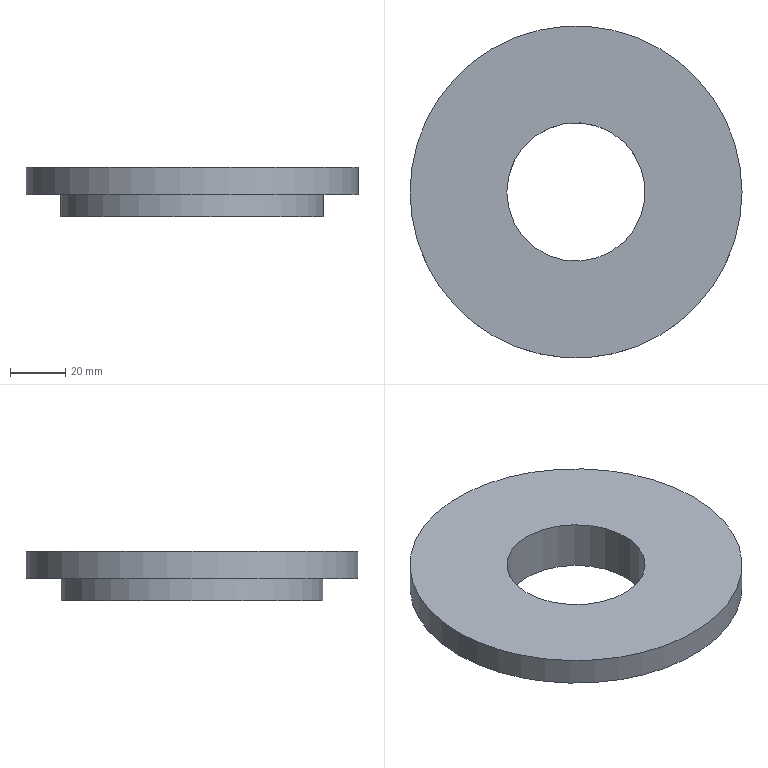Component | NX | COVER | 1 solid | 6 faces | box 120 x 120 x 18 mm | volume 134460 mm3 | plane 3 | cylinder 3 | commonest cylinder face diameters 120 x1 95 x1 50 x1
STEP:
#1=CARTESIAN_POINT('',(0.,0.,0.));
#2=DIRECTION('',(0.,0.,1.));
#3=DIRECTION('',(1.,0.,0.));
#4=AXIS2_PLACEMENT_3D('',#1,#2,#3);
#5=CARTESIAN_POINT('',(-449.175,308.181,125.));
#6=VERTEX_POINT('',#5);
#7=CARTESIAN_POINT('',(-424.175,308.181,125.));
#8=DIRECTION('',(0.,0.,-1.));
#9=DIRECTION('',(-1.,0.,0.));
#10=AXIS2_PLACEMENT_3D('',#7,#8,#9);
#11=CIRCLE('',#10,25.);
#12=CARTESIAN_POINT('',(-424.175,308.181,125.));
#13=DIRECTION('',(0.,0.,1.));
#14=DIRECTION('',(1.,0.,0.));
#15=AXIS2_PLACEMENT_3D('',#12,#13,#14);
#16=PLANE('',#15);
#17=CARTESIAN_POINT('',(-25.,0.));
#18=CARTESIAN_POINT('',(-25.,43.301));
#19=CARTESIAN_POINT('',(12.5,21.651));
#20=CARTESIAN_POINT('',(50.,0.));
#21=CARTESIAN_POINT('',(12.5,-21.651));
#22=CARTESIAN_POINT('',(-25.,-43.301));
#23=CARTESIAN_POINT('',(-25.,0.));
#24=(BOUNDED_CURVE()B_SPLINE_CURVE(2,(#17,#18,#19,#20,#21,#22,#23),.UNSPECIFIED.,.T.,.F.)B_SPLINE_CURVE_WITH_KNOTS((1,2,2,2,2,1),(-2.094,0.,2.094,4.189,6.283,8.378),.UNSPECIFIED.)CURVE()GEOMETRIC_REPRESENTATION_ITEM()RATIONAL_B_SPLINE_CURVE((1.,0.5,1.,0.5,1.,0.5,1.))REPRESENTATION_ITEM(''));
#25=(GEOMETRIC_REPRESENTATION_CONTEXT(2)PARAMETRIC_REPRESENTATION_CONTEXT()REPRESENTATION_CONTEXT('',''));
#26=DEFINITIONAL_REPRESENTATION('',(#24),#25);
#27=PCURVE('',#16,#26);
#28=CARTESIAN_POINT('',(-424.175,308.181,125.));
#29=DIRECTION('',(0.,0.,-1.));
#30=DIRECTION('',(-1.,0.,0.));
#31=AXIS2_PLACEMENT_3D('',#28,#29,#30);
#32=CYLINDRICAL_SURFACE('',#31,25.);
#33=CARTESIAN_POINT('',(0.,0.));
#34=DIRECTION('',(1.,0.));
#35=VECTOR('',#34,1.);
#36=LINE('',#33,#35);
#37=(GEOMETRIC_REPRESENTATION_CONTEXT(2)PARAMETRIC_REPRESENTATION_CONTEXT()REPRESENTATION_CONTEXT('',''));
#38=DEFINITIONAL_REPRESENTATION('',(#36),#37);
#39=PCURVE('',#32,#38);
#40=SURFACE_CURVE('',#11,(#27,#39),.PCURVE_S1.);
#41=EDGE_CURVE('',#6,#6,#40,.T.);
#42=ORIENTED_EDGE('',*,*,#41,.T.);
#43=EDGE_LOOP('',(#42));
#44=FACE_BOUND('',#43,.T.);
#45=CARTESIAN_POINT('',(-364.175,308.181,125.));
#46=VERTEX_POINT('',#45);
#47=CARTESIAN_POINT('',(-424.175,308.181,125.));
#48=DIRECTION('',(0.,0.,-1.));
#49=DIRECTION('',(1.,0.,0.));
#50=AXIS2_PLACEMENT_3D('',#47,#48,#49);
#51=CIRCLE('',#50,60.);
#52=CARTESIAN_POINT('',(60.,0.));
#53=CARTESIAN_POINT('',(60.,-103.923));
#54=CARTESIAN_POINT('',(-30.,-51.962));
#55=CARTESIAN_POINT('',(-120.,-0.));
#56=CARTESIAN_POINT('',(-30.,51.962));
#57=CARTESIAN_POINT('',(60.,103.923));
#58=CARTESIAN_POINT('',(60.,0.));
#59=(BOUNDED_CURVE()B_SPLINE_CURVE(2,(#52,#53,#54,#55,#56,#57,#58),.UNSPECIFIED.,.T.,.F.)B_SPLINE_CURVE_WITH_KNOTS((1,2,2,2,2,1),(-2.094,0.,2.094,4.189,6.283,8.378),.UNSPECIFIED.)CURVE()GEOMETRIC_REPRESENTATION_ITEM()RATIONAL_B_SPLINE_CURVE((1.,0.5,1.,0.5,1.,0.5,1.))REPRESENTATION_ITEM(''));
#60=(GEOMETRIC_REPRESENTATION_CONTEXT(2)PARAMETRIC_REPRESENTATION_CONTEXT()REPRESENTATION_CONTEXT('',''));
#61=DEFINITIONAL_REPRESENTATION('',(#59),#60);
#62=PCURVE('',#16,#61);
#63=CARTESIAN_POINT('',(-424.175,308.181,115.));
#64=DIRECTION('',(0.,0.,1.));
#65=DIRECTION('',(1.,0.,0.));
#66=AXIS2_PLACEMENT_3D('',#63,#64,#65);
#67=CYLINDRICAL_SURFACE('',#66,60.);
#68=CARTESIAN_POINT('',(6.283,10.));
#69=DIRECTION('',(-1.,0.));
#70=VECTOR('',#69,1.);
#71=LINE('',#68,#70);
#72=(GEOMETRIC_REPRESENTATION_CONTEXT(2)PARAMETRIC_REPRESENTATION_CONTEXT()REPRESENTATION_CONTEXT('',''));
#73=DEFINITIONAL_REPRESENTATION('',(#71),#72);
#74=PCURVE('',#67,#73);
#75=SURFACE_CURVE('',#51,(#62,#74),.PCURVE_S1.);
#76=EDGE_CURVE('',#46,#46,#75,.T.);
#77=ORIENTED_EDGE('',*,*,#76,.F.);
#78=EDGE_LOOP('',(#77));
#79=FACE_BOUND('',#78,.T.);
#80=ADVANCED_FACE('',(#44,#79),#16,.T.);
#81=CARTESIAN_POINT('',(-471.675,308.181,115.));
#82=VERTEX_POINT('',#81);
#83=CARTESIAN_POINT('',(-376.675,308.181,115.));
#84=VERTEX_POINT('',#83);
#85=CARTESIAN_POINT('',(-424.175,308.181,115.));
#86=DIRECTION('',(0.,0.,-1.));
#87=DIRECTION('',(-1.,0.,0.));
#88=AXIS2_PLACEMENT_3D('',#85,#86,#87);
#89=CIRCLE('',#88,47.5);
#90=CARTESIAN_POINT('',(-424.175,308.181,115.));
#91=DIRECTION('',(0.,0.,-1.));
#92=DIRECTION('',(-1.,0.,0.));
#93=AXIS2_PLACEMENT_3D('',#90,#91,#92);
#94=PLANE('',#93);
#95=CARTESIAN_POINT('',(0.,0.));
#96=DIRECTION('',(1.,0.));
#97=AXIS2_PLACEMENT_2D('',#95,#96);
#98=CIRCLE('',#97,47.5);
#99=(GEOMETRIC_REPRESENTATION_CONTEXT(2)PARAMETRIC_REPRESENTATION_CONTEXT()REPRESENTATION_CONTEXT('',''));
#100=DEFINITIONAL_REPRESENTATION('',(#98),#99);
#101=PCURVE('',#94,#100);
#102=CARTESIAN_POINT('',(-424.175,308.181,115.));
#103=DIRECTION('',(0.,0.,-1.));
#104=DIRECTION('',(1.,0.,0.));
#105=AXIS2_PLACEMENT_3D('',#102,#103,#104);
#106=CYLINDRICAL_SURFACE('',#105,47.5);
#107=CARTESIAN_POINT('',(3.142,0.));
#108=DIRECTION('',(1.,0.));
#109=VECTOR('',#108,1.);
#110=LINE('',#107,#109);
#111=(GEOMETRIC_REPRESENTATION_CONTEXT(2)PARAMETRIC_REPRESENTATION_CONTEXT()REPRESENTATION_CONTEXT('',''));
#112=DEFINITIONAL_REPRESENTATION('',(#110),#111);
#113=PCURVE('',#106,#112);
#114=SURFACE_CURVE('',#89,(#101,#113),.PCURVE_S1.);
#115=EDGE_CURVE('',#82,#84,#114,.T.);
#116=ORIENTED_EDGE('',*,*,#115,.F.);
#117=CARTESIAN_POINT('',(-424.175,308.181,115.));
#118=DIRECTION('',(0.,0.,-1.));
#119=DIRECTION('',(-1.,0.,0.));
#120=AXIS2_PLACEMENT_3D('',#117,#118,#119);
#121=CIRCLE('',#120,47.5);
#122=CARTESIAN_POINT('',(0.,0.));
#123=DIRECTION('',(1.,0.));
#124=AXIS2_PLACEMENT_2D('',#122,#123);
#125=CIRCLE('',#124,47.5);
#126=(GEOMETRIC_REPRESENTATION_CONTEXT(2)PARAMETRIC_REPRESENTATION_CONTEXT()REPRESENTATION_CONTEXT('',''));
#127=DEFINITIONAL_REPRESENTATION('',(#125),#126);
#128=PCURVE('',#94,#127);
#129=CARTESIAN_POINT('',(-3.142,0.));
#130=DIRECTION('',(1.,0.));
#131=VECTOR('',#130,1.);
#132=LINE('',#129,#131);
#133=(GEOMETRIC_REPRESENTATION_CONTEXT(2)PARAMETRIC_REPRESENTATION_CONTEXT()REPRESENTATION_CONTEXT('',''));
#134=DEFINITIONAL_REPRESENTATION('',(#132),#133);
#135=PCURVE('',#106,#134);
#136=SURFACE_CURVE('',#121,(#128,#135),.PCURVE_S1.);
#137=EDGE_CURVE('',#84,#82,#136,.T.);
#138=ORIENTED_EDGE('',*,*,#137,.F.);
#139=EDGE_LOOP('',(#116,#138));
#140=FACE_BOUND('',#139,.T.);
#141=CARTESIAN_POINT('',(-364.175,308.181,115.));
#142=VERTEX_POINT('',#141);
#143=CARTESIAN_POINT('',(-424.175,308.181,115.));
#144=DIRECTION('',(0.,0.,1.));
#145=DIRECTION('',(1.,0.,0.));
#146=AXIS2_PLACEMENT_3D('',#143,#144,#145);
#147=CIRCLE('',#146,60.);
#148=CARTESIAN_POINT('',(-60.,0.));
#149=CARTESIAN_POINT('',(-60.,103.923));
#150=CARTESIAN_POINT('',(30.,51.962));
#151=CARTESIAN_POINT('',(120.,0.));
#152=CARTESIAN_POINT('',(30.,-51.962));
#153=CARTESIAN_POINT('',(-60.,-103.923));
#154=CARTESIAN_POINT('',(-60.,0.));
#155=(BOUNDED_CURVE()B_SPLINE_CURVE(2,(#148,#149,#150,#151,#152,#153,#154),.UNSPECIFIED.,.T.,.F.)B_SPLINE_CURVE_WITH_KNOTS((1,2,2,2,2,1),(-2.094,0.,2.094,4.189,6.283,8.378),.UNSPECIFIED.)CURVE()GEOMETRIC_REPRESENTATION_ITEM()RATIONAL_B_SPLINE_CURVE((1.,0.5,1.,0.5,1.,0.5,1.))REPRESENTATION_ITEM(''));
#156=(GEOMETRIC_REPRESENTATION_CONTEXT(2)PARAMETRIC_REPRESENTATION_CONTEXT()REPRESENTATION_CONTEXT('',''));
#157=DEFINITIONAL_REPRESENTATION('',(#155),#156);
#158=PCURVE('',#94,#157);
#159=CARTESIAN_POINT('',(0.,0.));
#160=DIRECTION('',(1.,0.));
#161=VECTOR('',#160,1.);
#162=LINE('',#159,#161);
#163=(GEOMETRIC_REPRESENTATION_CONTEXT(2)PARAMETRIC_REPRESENTATION_CONTEXT()REPRESENTATION_CONTEXT('',''));
#164=DEFINITIONAL_REPRESENTATION('',(#162),#163);
#165=PCURVE('',#67,#164);
#166=SURFACE_CURVE('',#147,(#158,#165),.PCURVE_S1.);
#167=EDGE_CURVE('',#142,#142,#166,.T.);
#168=ORIENTED_EDGE('',*,*,#167,.F.);
#169=EDGE_LOOP('',(#168));
#170=FACE_BOUND('',#169,.T.);
#171=ADVANCED_FACE('',(#140,#170),#94,.T.);
#172=ORIENTED_EDGE('',*,*,#76,.T.);
#173=CARTESIAN_POINT('',(-364.175,308.181,115.));
#174=CARTESIAN_POINT('',(-364.175,308.181,125.));
#175=B_SPLINE_CURVE_WITH_KNOTS('',1,(#173,#174),.UNSPECIFIED.,.F.,.F.,(2,2),(0.,10.),.PIECEWISE_BEZIER_KNOTS.);
#176=CARTESIAN_POINT('',(0.,0.));
#177=DIRECTION('',(0.,1.));
#178=VECTOR('',#177,1.);
#179=LINE('',#176,#178);
#180=(GEOMETRIC_REPRESENTATION_CONTEXT(2)PARAMETRIC_REPRESENTATION_CONTEXT()REPRESENTATION_CONTEXT('',''));
#181=DEFINITIONAL_REPRESENTATION('',(#179),#180);
#182=PCURVE('',#67,#181);
#183=CARTESIAN_POINT('',(6.283,0.));
#184=DIRECTION('',(0.,1.));
#185=VECTOR('',#184,1.);
#186=LINE('',#183,#185);
#187=(GEOMETRIC_REPRESENTATION_CONTEXT(2)PARAMETRIC_REPRESENTATION_CONTEXT()REPRESENTATION_CONTEXT('',''));
#188=DEFINITIONAL_REPRESENTATION('',(#186),#187);
#189=PCURVE('',#67,#188);
#190=SEAM_CURVE('',#175,(#182,#189),.PCURVE_S1.);
#191=EDGE_CURVE('',#142,#46,#190,.T.);
#192=ORIENTED_EDGE('',*,*,#191,.F.);
#193=ORIENTED_EDGE('',*,*,#167,.T.);
#194=ORIENTED_EDGE('',*,*,#191,.T.);
#195=EDGE_LOOP('',(#172,#192,#193,#194));
#196=FACE_BOUND('',#195,.T.);
#197=ADVANCED_FACE('',(#196),#67,.T.);
#198=CARTESIAN_POINT('',(-449.175,308.181,107.));
#199=VERTEX_POINT('',#198);
#200=CARTESIAN_POINT('',(-424.175,308.181,107.));
#201=DIRECTION('',(0.,0.,-1.));
#202=DIRECTION('',(-1.,0.,0.));
#203=AXIS2_PLACEMENT_3D('',#200,#201,#202);
#204=CIRCLE('',#203,25.);
#205=CARTESIAN_POINT('',(-424.175,308.181,107.));
#206=DIRECTION('',(0.,0.,-1.));
#207=DIRECTION('',(-1.,0.,0.));
#208=AXIS2_PLACEMENT_3D('',#205,#206,#207);
#209=PLANE('',#208);
#210=CARTESIAN_POINT('',(0.,0.));
#211=DIRECTION('',(1.,0.));
#212=AXIS2_PLACEMENT_2D('',#210,#211);
#213=CIRCLE('',#212,25.);
#214=(GEOMETRIC_REPRESENTATION_CONTEXT(2)PARAMETRIC_REPRESENTATION_CONTEXT()REPRESENTATION_CONTEXT('',''));
#215=DEFINITIONAL_REPRESENTATION('',(#213),#214);
#216=PCURVE('',#209,#215);
#217=CARTESIAN_POINT('',(0.,18.));
#218=DIRECTION('',(1.,0.));
#219=VECTOR('',#218,1.);
#220=LINE('',#217,#219);
#221=(GEOMETRIC_REPRESENTATION_CONTEXT(2)PARAMETRIC_REPRESENTATION_CONTEXT()REPRESENTATION_CONTEXT('',''));
#222=DEFINITIONAL_REPRESENTATION('',(#220),#221);
#223=PCURVE('',#32,#222);
#224=SURFACE_CURVE('',#204,(#216,#223),.PCURVE_S1.);
#225=EDGE_CURVE('',#199,#199,#224,.T.);
#226=ORIENTED_EDGE('',*,*,#225,.F.);
#227=EDGE_LOOP('',(#226));
#228=FACE_BOUND('',#227,.T.);
#229=CARTESIAN_POINT('',(-376.675,308.181,107.));
#230=VERTEX_POINT('',#229);
#231=CARTESIAN_POINT('',(-424.175,308.181,107.));
#232=DIRECTION('',(0.,0.,1.));
#233=DIRECTION('',(1.,0.,0.));
#234=AXIS2_PLACEMENT_3D('',#231,#232,#233);
#235=CIRCLE('',#234,47.5);
#236=CARTESIAN_POINT('',(-47.5,0.));
#237=CARTESIAN_POINT('',(-47.5,82.272));
#238=CARTESIAN_POINT('',(23.75,41.136));
#239=CARTESIAN_POINT('',(95.,0.));
#240=CARTESIAN_POINT('',(23.75,-41.136));
#241=CARTESIAN_POINT('',(-47.5,-82.272));
#242=CARTESIAN_POINT('',(-47.5,0.));
#243=(BOUNDED_CURVE()B_SPLINE_CURVE(2,(#236,#237,#238,#239,#240,#241,#242),.UNSPECIFIED.,.T.,.F.)B_SPLINE_CURVE_WITH_KNOTS((1,2,2,2,2,1),(-2.094,0.,2.094,4.189,6.283,8.378),.UNSPECIFIED.)CURVE()GEOMETRIC_REPRESENTATION_ITEM()RATIONAL_B_SPLINE_CURVE((1.,0.5,1.,0.5,1.,0.5,1.))REPRESENTATION_ITEM(''));
#244=(GEOMETRIC_REPRESENTATION_CONTEXT(2)PARAMETRIC_REPRESENTATION_CONTEXT()REPRESENTATION_CONTEXT('',''));
#245=DEFINITIONAL_REPRESENTATION('',(#243),#244);
#246=PCURVE('',#209,#245);
#247=CARTESIAN_POINT('',(6.283,8.));
#248=DIRECTION('',(-1.,0.));
#249=VECTOR('',#248,1.);
#250=LINE('',#247,#249);
#251=(GEOMETRIC_REPRESENTATION_CONTEXT(2)PARAMETRIC_REPRESENTATION_CONTEXT()REPRESENTATION_CONTEXT('',''));
#252=DEFINITIONAL_REPRESENTATION('',(#250),#251);
#253=PCURVE('',#106,#252);
#254=SURFACE_CURVE('',#235,(#246,#253),.PCURVE_S1.);
#255=EDGE_CURVE('',#230,#230,#254,.T.);
#256=ORIENTED_EDGE('',*,*,#255,.F.);
#257=EDGE_LOOP('',(#256));
#258=FACE_BOUND('',#257,.T.);
#259=ADVANCED_FACE('',(#228,#258),#209,.T.);
#260=ORIENTED_EDGE('',*,*,#255,.T.);
#261=CARTESIAN_POINT('',(-376.675,308.181,115.));
#262=CARTESIAN_POINT('',(-376.675,308.181,107.));
#263=B_SPLINE_CURVE_WITH_KNOTS('',1,(#261,#262),.UNSPECIFIED.,.F.,.F.,(2,2),(0.,8.),.PIECEWISE_BEZIER_KNOTS.);
#264=CARTESIAN_POINT('',(0.,0.));
#265=DIRECTION('',(0.,1.));
#266=VECTOR('',#265,1.);
#267=LINE('',#264,#266);
#268=(GEOMETRIC_REPRESENTATION_CONTEXT(2)PARAMETRIC_REPRESENTATION_CONTEXT()REPRESENTATION_CONTEXT('',''));
#269=DEFINITIONAL_REPRESENTATION('',(#267),#268);
#270=PCURVE('',#106,#269);
#271=CARTESIAN_POINT('',(6.283,0.));
#272=DIRECTION('',(0.,1.));
#273=VECTOR('',#272,1.);
#274=LINE('',#271,#273);
#275=(GEOMETRIC_REPRESENTATION_CONTEXT(2)PARAMETRIC_REPRESENTATION_CONTEXT()REPRESENTATION_CONTEXT('',''));
#276=DEFINITIONAL_REPRESENTATION('',(#274),#275);
#277=PCURVE('',#106,#276);
#278=SEAM_CURVE('',#263,(#270,#277),.PCURVE_S1.);
#279=EDGE_CURVE('',#84,#230,#278,.T.);
#280=ORIENTED_EDGE('',*,*,#279,.F.);
#281=ORIENTED_EDGE('',*,*,#137,.T.);
#282=ORIENTED_EDGE('',*,*,#115,.T.);
#283=ORIENTED_EDGE('',*,*,#279,.T.);
#284=EDGE_LOOP('',(#260,#280,#281,#282,#283));
#285=FACE_BOUND('',#284,.T.);
#286=ADVANCED_FACE('',(#285),#106,.T.);
#287=ORIENTED_EDGE('',*,*,#225,.F.);
#288=CARTESIAN_POINT('',(-449.175,308.181,125.));
#289=CARTESIAN_POINT('',(-449.175,308.181,107.));
#290=B_SPLINE_CURVE_WITH_KNOTS('',1,(#288,#289),.UNSPECIFIED.,.F.,.F.,(2,2),(0.,18.),.PIECEWISE_BEZIER_KNOTS.);
#291=CARTESIAN_POINT('',(0.,0.));
#292=DIRECTION('',(0.,1.));
#293=VECTOR('',#292,1.);
#294=LINE('',#291,#293);
#295=(GEOMETRIC_REPRESENTATION_CONTEXT(2)PARAMETRIC_REPRESENTATION_CONTEXT()REPRESENTATION_CONTEXT('',''));
#296=DEFINITIONAL_REPRESENTATION('',(#294),#295);
#297=PCURVE('',#32,#296);
#298=CARTESIAN_POINT('',(6.283,0.));
#299=DIRECTION('',(0.,1.));
#300=VECTOR('',#299,1.);
#301=LINE('',#298,#300);
#302=(GEOMETRIC_REPRESENTATION_CONTEXT(2)PARAMETRIC_REPRESENTATION_CONTEXT()REPRESENTATION_CONTEXT('',''));
#303=DEFINITIONAL_REPRESENTATION('',(#301),#302);
#304=PCURVE('',#32,#303);
#305=SEAM_CURVE('',#290,(#297,#304),.PCURVE_S1.);
#306=EDGE_CURVE('',#6,#199,#305,.T.);
#307=ORIENTED_EDGE('',*,*,#306,.F.);
#308=ORIENTED_EDGE('',*,*,#41,.T.);
#309=ORIENTED_EDGE('',*,*,#306,.T.);
#310=EDGE_LOOP('',(#287,#307,#308,#309));
#311=FACE_BOUND('',#310,.F.);
#312=ADVANCED_FACE('',(#311),#32,.F.);
#313=CLOSED_SHELL('',(#80,#171,#197,#259,#286,#312));
#314=MANIFOLD_SOLID_BREP('',#313);
#315=(LENGTH_UNIT()NAMED_UNIT(*)SI_UNIT(.MILLI.,.METRE.));
#316=UNCERTAINTY_MEASURE_WITH_UNIT(LENGTH_MEASURE(0.000005),#315,'','');
#317=(NAMED_UNIT(*)PLANE_ANGLE_UNIT()SI_UNIT($,.RADIAN.));
#318=(NAMED_UNIT(*)SI_UNIT($,.STERADIAN.)SOLID_ANGLE_UNIT());
#319=(GEOMETRIC_REPRESENTATION_CONTEXT(3)GLOBAL_UNCERTAINTY_ASSIGNED_CONTEXT((#316))GLOBAL_UNIT_ASSIGNED_CONTEXT((#315,#317,#318))REPRESENTATION_CONTEXT('',''));
#320=ADVANCED_BREP_SHAPE_REPRESENTATION('',(#4,#314),#319);